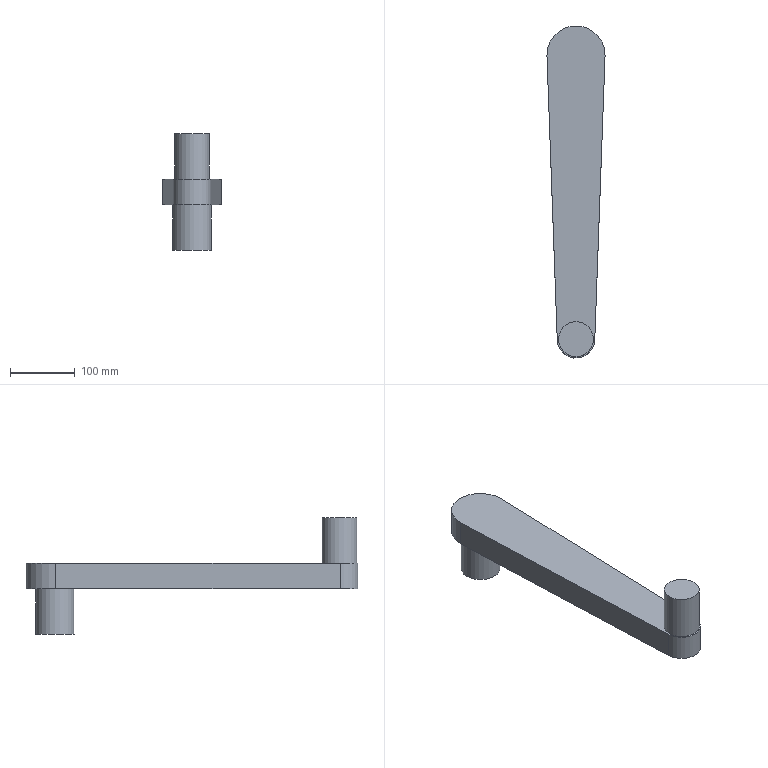Component | NX | PART_3 | 1 solid | 10 faces | box 90 x 514.09 x 180 mm | volume 1841830 mm3 | plane 6 | cylinder 4 | commonest cylinder face diameters 58 x1 90 x1 54 x1 60 x1
STEP:
#1=CARTESIAN_POINT('',(0.,0.,0.));
#2=DIRECTION('',(0.,0.,1.));
#3=DIRECTION('',(1.,0.,0.));
#4=AXIS2_PLACEMENT_3D('',#1,#2,#3);
#5=CARTESIAN_POINT('',(-201.014,-230.518,0.));
#6=VERTEX_POINT('',#5);
#7=CARTESIAN_POINT('',(-185.024,-670.023,0.));
#8=VERTEX_POINT('',#7);
#9=CARTESIAN_POINT('',(-201.014,-230.518,0.));
#10=DIRECTION('',(0.03636,-0.9993,0.));
#11=VECTOR('',#10,1.);
#12=LINE('',#9,#11);
#13=CARTESIAN_POINT('',(-201.014,-230.518,40.));
#14=DIRECTION('',(0.9993,0.03636,0.));
#15=DIRECTION('',(-0.03636,0.9993,0.));
#16=AXIS2_PLACEMENT_3D('',#13,#14,#15);
#17=PLANE('',#16);
#18=CARTESIAN_POINT('',(0.,-40.));
#19=DIRECTION('',(-1.,0.));
#20=VECTOR('',#19,1.);
#21=LINE('',#18,#20);
#22=(GEOMETRIC_REPRESENTATION_CONTEXT(2)PARAMETRIC_REPRESENTATION_CONTEXT()REPRESENTATION_CONTEXT('',''));
#23=DEFINITIONAL_REPRESENTATION('',(#21),#22);
#24=PCURVE('',#17,#23);
#25=CARTESIAN_POINT('',(-156.043,-668.969,0.));
#26=DIRECTION('',(0.,0.,1.));
#27=DIRECTION('',(1.,0.,0.));
#28=AXIS2_PLACEMENT_3D('',#25,#26,#27);
#29=PLANE('',#28);
#30=CARTESIAN_POINT('',(-44.97,438.451));
#31=DIRECTION('',(0.03636,-0.9993));
#32=VECTOR('',#31,1.);
#33=LINE('',#30,#32);
#34=(GEOMETRIC_REPRESENTATION_CONTEXT(2)PARAMETRIC_REPRESENTATION_CONTEXT()REPRESENTATION_CONTEXT('',''));
#35=DEFINITIONAL_REPRESENTATION('',(#33),#34);
#36=PCURVE('',#29,#35);
#37=SURFACE_CURVE('',#12,(#24,#36),.PCURVE_S1.);
#38=EDGE_CURVE('',#6,#8,#37,.T.);
#39=ORIENTED_EDGE('',*,*,#38,.T.);
#40=CARTESIAN_POINT('',(-185.024,-670.023,40.));
#41=VERTEX_POINT('',#40);
#42=CARTESIAN_POINT('',(-185.024,-670.023,40.));
#43=DIRECTION('',(0.,0.,-1.));
#44=VECTOR('',#43,1.);
#45=LINE('',#42,#44);
#46=CARTESIAN_POINT('',(-439.796,0.));
#47=DIRECTION('',(0.,-1.));
#48=VECTOR('',#47,1.);
#49=LINE('',#46,#48);
#50=(GEOMETRIC_REPRESENTATION_CONTEXT(2)PARAMETRIC_REPRESENTATION_CONTEXT()REPRESENTATION_CONTEXT('',''));
#51=DEFINITIONAL_REPRESENTATION('',(#49),#50);
#52=PCURVE('',#17,#51);
#53=CARTESIAN_POINT('',(-156.043,-668.969,40.));
#54=DIRECTION('',(0.,0.,-1.));
#55=DIRECTION('',(-1.,0.,0.));
#56=AXIS2_PLACEMENT_3D('',#53,#54,#55);
#57=CYLINDRICAL_SURFACE('',#56,29.);
#58=CARTESIAN_POINT('',(6.247,0.));
#59=DIRECTION('',(0.,1.));
#60=VECTOR('',#59,1.);
#61=LINE('',#58,#60);
#62=(GEOMETRIC_REPRESENTATION_CONTEXT(2)PARAMETRIC_REPRESENTATION_CONTEXT()REPRESENTATION_CONTEXT('',''));
#63=DEFINITIONAL_REPRESENTATION('',(#61),#62);
#64=PCURVE('',#57,#63);
#65=SURFACE_CURVE('',#45,(#52,#64),.PCURVE_S1.);
#66=EDGE_CURVE('',#41,#8,#65,.T.);
#67=ORIENTED_EDGE('',*,*,#66,.F.);
#68=CARTESIAN_POINT('',(-201.014,-230.518,40.));
#69=VERTEX_POINT('',#68);
#70=CARTESIAN_POINT('',(-201.014,-230.518,40.));
#71=DIRECTION('',(0.03636,-0.9993,0.));
#72=VECTOR('',#71,1.);
#73=LINE('',#70,#72);
#74=CARTESIAN_POINT('',(0.,0.));
#75=DIRECTION('',(-1.,0.));
#76=VECTOR('',#75,1.);
#77=LINE('',#74,#76);
#78=(GEOMETRIC_REPRESENTATION_CONTEXT(2)PARAMETRIC_REPRESENTATION_CONTEXT()REPRESENTATION_CONTEXT('',''));
#79=DEFINITIONAL_REPRESENTATION('',(#77),#78);
#80=PCURVE('',#17,#79);
#81=CARTESIAN_POINT('',(-156.043,-668.969,40.));
#82=DIRECTION('',(0.,0.,1.));
#83=DIRECTION('',(1.,0.,0.));
#84=AXIS2_PLACEMENT_3D('',#81,#82,#83);
#85=PLANE('',#84);
#86=CARTESIAN_POINT('',(-44.97,438.451));
#87=DIRECTION('',(0.03636,-0.9993));
#88=VECTOR('',#87,1.);
#89=LINE('',#86,#88);
#90=(GEOMETRIC_REPRESENTATION_CONTEXT(2)PARAMETRIC_REPRESENTATION_CONTEXT()REPRESENTATION_CONTEXT('',''));
#91=DEFINITIONAL_REPRESENTATION('',(#89),#90);
#92=PCURVE('',#85,#91);
#93=SURFACE_CURVE('',#73,(#80,#92),.PCURVE_S1.);
#94=EDGE_CURVE('',#69,#41,#93,.T.);
#95=ORIENTED_EDGE('',*,*,#94,.F.);
#96=CARTESIAN_POINT('',(-201.014,-230.518,40.));
#97=DIRECTION('',(0.,0.,-1.));
#98=VECTOR('',#97,1.);
#99=LINE('',#96,#98);
#100=CARTESIAN_POINT('',(0.,0.));
#101=DIRECTION('',(0.,-1.));
#102=VECTOR('',#101,1.);
#103=LINE('',#100,#102);
#104=(GEOMETRIC_REPRESENTATION_CONTEXT(2)PARAMETRIC_REPRESENTATION_CONTEXT()REPRESENTATION_CONTEXT('',''));
#105=DEFINITIONAL_REPRESENTATION('',(#103),#104);
#106=PCURVE('',#17,#105);
#107=CARTESIAN_POINT('',(-156.043,-228.882,40.));
#108=DIRECTION('',(0.,0.,-1.));
#109=DIRECTION('',(-1.,0.,0.));
#110=AXIS2_PLACEMENT_3D('',#107,#108,#109);
#111=CYLINDRICAL_SURFACE('',#110,45.);
#112=CARTESIAN_POINT('',(-0.03636,0.));
#113=DIRECTION('',(0.,1.));
#114=VECTOR('',#113,1.);
#115=LINE('',#112,#114);
#116=(GEOMETRIC_REPRESENTATION_CONTEXT(2)PARAMETRIC_REPRESENTATION_CONTEXT()REPRESENTATION_CONTEXT('',''));
#117=DEFINITIONAL_REPRESENTATION('',(#115),#116);
#118=PCURVE('',#111,#117);
#119=SURFACE_CURVE('',#99,(#106,#118),.PCURVE_S1.);
#120=EDGE_CURVE('',#69,#6,#119,.T.);
#121=ORIENTED_EDGE('',*,*,#120,.T.);
#122=EDGE_LOOP('',(#39,#67,#95,#121));
#123=FACE_BOUND('',#122,.T.);
#124=ADVANCED_FACE('',(#123),#17,.F.);
#125=CARTESIAN_POINT('',(-127.062,-670.023,0.));
#126=VERTEX_POINT('',#125);
#127=CARTESIAN_POINT('',(-156.043,-668.969,0.));
#128=DIRECTION('',(0.,0.,1.));
#129=DIRECTION('',(1.,0.,0.));
#130=AXIS2_PLACEMENT_3D('',#127,#128,#129);
#131=CIRCLE('',#130,29.);
#132=CARTESIAN_POINT('',(9.425,40.));
#133=DIRECTION('',(-1.,0.));
#134=VECTOR('',#133,1.);
#135=LINE('',#132,#134);
#136=(GEOMETRIC_REPRESENTATION_CONTEXT(2)PARAMETRIC_REPRESENTATION_CONTEXT()REPRESENTATION_CONTEXT('',''));
#137=DEFINITIONAL_REPRESENTATION('',(#135),#136);
#138=PCURVE('',#57,#137);
#139=CARTESIAN_POINT('',(0.,0.));
#140=DIRECTION('',(1.,0.));
#141=AXIS2_PLACEMENT_2D('',#139,#140);
#142=CIRCLE('',#141,29.);
#143=(GEOMETRIC_REPRESENTATION_CONTEXT(2)PARAMETRIC_REPRESENTATION_CONTEXT()REPRESENTATION_CONTEXT('',''));
#144=DEFINITIONAL_REPRESENTATION('',(#142),#143);
#145=PCURVE('',#29,#144);
#146=SURFACE_CURVE('',#131,(#138,#145),.PCURVE_S1.);
#147=EDGE_CURVE('',#8,#126,#146,.T.);
#148=ORIENTED_EDGE('',*,*,#147,.T.);
#149=CARTESIAN_POINT('',(-127.062,-670.023,40.));
#150=VERTEX_POINT('',#149);
#151=CARTESIAN_POINT('',(-127.062,-670.023,40.));
#152=DIRECTION('',(0.,0.,-1.));
#153=VECTOR('',#152,1.);
#154=LINE('',#151,#153);
#155=CARTESIAN_POINT('',(3.178,0.));
#156=DIRECTION('',(0.,1.));
#157=VECTOR('',#156,1.);
#158=LINE('',#155,#157);
#159=(GEOMETRIC_REPRESENTATION_CONTEXT(2)PARAMETRIC_REPRESENTATION_CONTEXT()REPRESENTATION_CONTEXT('',''));
#160=DEFINITIONAL_REPRESENTATION('',(#158),#159);
#161=PCURVE('',#57,#160);
#162=CARTESIAN_POINT('',(-127.062,-670.023,40.));
#163=DIRECTION('',(-0.9993,0.03636,0.));
#164=DIRECTION('',(-0.03636,-0.9993,0.));
#165=AXIS2_PLACEMENT_3D('',#162,#163,#164);
#166=PLANE('',#165);
#167=CARTESIAN_POINT('',(0.,0.));
#168=DIRECTION('',(0.,-1.));
#169=VECTOR('',#168,1.);
#170=LINE('',#167,#169);
#171=(GEOMETRIC_REPRESENTATION_CONTEXT(2)PARAMETRIC_REPRESENTATION_CONTEXT()REPRESENTATION_CONTEXT('',''));
#172=DEFINITIONAL_REPRESENTATION('',(#170),#171);
#173=PCURVE('',#166,#172);
#174=SURFACE_CURVE('',#154,(#161,#173),.PCURVE_S1.);
#175=EDGE_CURVE('',#150,#126,#174,.T.);
#176=ORIENTED_EDGE('',*,*,#175,.F.);
#177=CARTESIAN_POINT('',(-156.043,-668.969,40.));
#178=DIRECTION('',(0.,0.,1.));
#179=DIRECTION('',(1.,0.,0.));
#180=AXIS2_PLACEMENT_3D('',#177,#178,#179);
#181=CIRCLE('',#180,29.);
#182=CARTESIAN_POINT('',(9.425,0.));
#183=DIRECTION('',(-1.,0.));
#184=VECTOR('',#183,1.);
#185=LINE('',#182,#184);
#186=(GEOMETRIC_REPRESENTATION_CONTEXT(2)PARAMETRIC_REPRESENTATION_CONTEXT()REPRESENTATION_CONTEXT('',''));
#187=DEFINITIONAL_REPRESENTATION('',(#185),#186);
#188=PCURVE('',#57,#187);
#189=CARTESIAN_POINT('',(0.,0.));
#190=DIRECTION('',(1.,0.));
#191=AXIS2_PLACEMENT_2D('',#189,#190);
#192=CIRCLE('',#191,29.);
#193=(GEOMETRIC_REPRESENTATION_CONTEXT(2)PARAMETRIC_REPRESENTATION_CONTEXT()REPRESENTATION_CONTEXT('',''));
#194=DEFINITIONAL_REPRESENTATION('',(#192),#193);
#195=PCURVE('',#85,#194);
#196=SURFACE_CURVE('',#181,(#188,#195),.PCURVE_S1.);
#197=EDGE_CURVE('',#41,#150,#196,.T.);
#198=ORIENTED_EDGE('',*,*,#197,.F.);
#199=ORIENTED_EDGE('',*,*,#66,.T.);
#200=EDGE_LOOP('',(#148,#176,#198,#199));
#201=FACE_BOUND('',#200,.T.);
#202=ADVANCED_FACE('',(#201),#57,.T.);
#203=CARTESIAN_POINT('',(-111.073,-230.518,0.));
#204=VERTEX_POINT('',#203);
#205=CARTESIAN_POINT('',(-127.062,-670.023,0.));
#206=DIRECTION('',(0.03636,0.9993,0.));
#207=VECTOR('',#206,1.);
#208=LINE('',#205,#207);
#209=CARTESIAN_POINT('',(0.,-40.));
#210=DIRECTION('',(-1.,0.));
#211=VECTOR('',#210,1.);
#212=LINE('',#209,#211);
#213=(GEOMETRIC_REPRESENTATION_CONTEXT(2)PARAMETRIC_REPRESENTATION_CONTEXT()REPRESENTATION_CONTEXT('',''));
#214=DEFINITIONAL_REPRESENTATION('',(#212),#213);
#215=PCURVE('',#166,#214);
#216=CARTESIAN_POINT('',(28.981,-1.054));
#217=DIRECTION('',(0.03636,0.9993));
#218=VECTOR('',#217,1.);
#219=LINE('',#216,#218);
#220=(GEOMETRIC_REPRESENTATION_CONTEXT(2)PARAMETRIC_REPRESENTATION_CONTEXT()REPRESENTATION_CONTEXT('',''));
#221=DEFINITIONAL_REPRESENTATION('',(#219),#220);
#222=PCURVE('',#29,#221);
#223=SURFACE_CURVE('',#208,(#215,#222),.PCURVE_S1.);
#224=EDGE_CURVE('',#126,#204,#223,.T.);
#225=ORIENTED_EDGE('',*,*,#224,.T.);
#226=CARTESIAN_POINT('',(-111.073,-230.518,40.));
#227=VERTEX_POINT('',#226);
#228=CARTESIAN_POINT('',(-111.073,-230.518,40.));
#229=DIRECTION('',(0.,0.,-1.));
#230=VECTOR('',#229,1.);
#231=LINE('',#228,#230);
#232=CARTESIAN_POINT('',(-439.796,0.));
#233=DIRECTION('',(0.,-1.));
#234=VECTOR('',#233,1.);
#235=LINE('',#232,#234);
#236=(GEOMETRIC_REPRESENTATION_CONTEXT(2)PARAMETRIC_REPRESENTATION_CONTEXT()REPRESENTATION_CONTEXT('',''));
#237=DEFINITIONAL_REPRESENTATION('',(#235),#236);
#238=PCURVE('',#166,#237);
#239=CARTESIAN_POINT('',(3.178,0.));
#240=DIRECTION('',(0.,1.));
#241=VECTOR('',#240,1.);
#242=LINE('',#239,#241);
#243=(GEOMETRIC_REPRESENTATION_CONTEXT(2)PARAMETRIC_REPRESENTATION_CONTEXT()REPRESENTATION_CONTEXT('',''));
#244=DEFINITIONAL_REPRESENTATION('',(#242),#243);
#245=PCURVE('',#111,#244);
#246=SURFACE_CURVE('',#231,(#238,#245),.PCURVE_S1.);
#247=EDGE_CURVE('',#227,#204,#246,.T.);
#248=ORIENTED_EDGE('',*,*,#247,.F.);
#249=CARTESIAN_POINT('',(-127.062,-670.023,40.));
#250=DIRECTION('',(0.03636,0.9993,0.));
#251=VECTOR('',#250,1.);
#252=LINE('',#249,#251);
#253=CARTESIAN_POINT('',(0.,0.));
#254=DIRECTION('',(-1.,0.));
#255=VECTOR('',#254,1.);
#256=LINE('',#253,#255);
#257=(GEOMETRIC_REPRESENTATION_CONTEXT(2)PARAMETRIC_REPRESENTATION_CONTEXT()REPRESENTATION_CONTEXT('',''));
#258=DEFINITIONAL_REPRESENTATION('',(#256),#257);
#259=PCURVE('',#166,#258);
#260=CARTESIAN_POINT('',(28.981,-1.054));
#261=DIRECTION('',(0.03636,0.9993));
#262=VECTOR('',#261,1.);
#263=LINE('',#260,#262);
#264=(GEOMETRIC_REPRESENTATION_CONTEXT(2)PARAMETRIC_REPRESENTATION_CONTEXT()REPRESENTATION_CONTEXT('',''));
#265=DEFINITIONAL_REPRESENTATION('',(#263),#264);
#266=PCURVE('',#85,#265);
#267=SURFACE_CURVE('',#252,(#259,#266),.PCURVE_S1.);
#268=EDGE_CURVE('',#150,#227,#267,.T.);
#269=ORIENTED_EDGE('',*,*,#268,.F.);
#270=ORIENTED_EDGE('',*,*,#175,.T.);
#271=EDGE_LOOP('',(#225,#248,#269,#270));
#272=FACE_BOUND('',#271,.T.);
#273=ADVANCED_FACE('',(#272),#166,.F.);
#274=CARTESIAN_POINT('',(-156.043,-228.882,0.));
#275=DIRECTION('',(0.,0.,1.));
#276=DIRECTION('',(1.,0.,0.));
#277=AXIS2_PLACEMENT_3D('',#274,#275,#276);
#278=CIRCLE('',#277,45.);
#279=CARTESIAN_POINT('',(9.425,40.));
#280=DIRECTION('',(-1.,0.));
#281=VECTOR('',#280,1.);
#282=LINE('',#279,#281);
#283=(GEOMETRIC_REPRESENTATION_CONTEXT(2)PARAMETRIC_REPRESENTATION_CONTEXT()REPRESENTATION_CONTEXT('',''));
#284=DEFINITIONAL_REPRESENTATION('',(#282),#283);
#285=PCURVE('',#111,#284);
#286=CARTESIAN_POINT('',(0.,440.087));
#287=DIRECTION('',(1.,0.));
#288=AXIS2_PLACEMENT_2D('',#286,#287);
#289=CIRCLE('',#288,45.);
#290=(GEOMETRIC_REPRESENTATION_CONTEXT(2)PARAMETRIC_REPRESENTATION_CONTEXT()REPRESENTATION_CONTEXT('',''));
#291=DEFINITIONAL_REPRESENTATION('',(#289),#290);
#292=PCURVE('',#29,#291);
#293=SURFACE_CURVE('',#278,(#285,#292),.PCURVE_S1.);
#294=EDGE_CURVE('',#204,#6,#293,.T.);
#295=ORIENTED_EDGE('',*,*,#294,.T.);
#296=ORIENTED_EDGE('',*,*,#120,.F.);
#297=CARTESIAN_POINT('',(-156.043,-228.882,40.));
#298=DIRECTION('',(0.,0.,1.));
#299=DIRECTION('',(1.,0.,0.));
#300=AXIS2_PLACEMENT_3D('',#297,#298,#299);
#301=CIRCLE('',#300,45.);
#302=CARTESIAN_POINT('',(9.425,0.));
#303=DIRECTION('',(-1.,0.));
#304=VECTOR('',#303,1.);
#305=LINE('',#302,#304);
#306=(GEOMETRIC_REPRESENTATION_CONTEXT(2)PARAMETRIC_REPRESENTATION_CONTEXT()REPRESENTATION_CONTEXT('',''));
#307=DEFINITIONAL_REPRESENTATION('',(#305),#306);
#308=PCURVE('',#111,#307);
#309=CARTESIAN_POINT('',(0.,440.087));
#310=DIRECTION('',(1.,0.));
#311=AXIS2_PLACEMENT_2D('',#309,#310);
#312=CIRCLE('',#311,45.);
#313=(GEOMETRIC_REPRESENTATION_CONTEXT(2)PARAMETRIC_REPRESENTATION_CONTEXT()REPRESENTATION_CONTEXT('',''));
#314=DEFINITIONAL_REPRESENTATION('',(#312),#313);
#315=PCURVE('',#85,#314);
#316=SURFACE_CURVE('',#301,(#308,#315),.PCURVE_S1.);
#317=EDGE_CURVE('',#227,#69,#316,.T.);
#318=ORIENTED_EDGE('',*,*,#317,.F.);
#319=ORIENTED_EDGE('',*,*,#247,.T.);
#320=EDGE_LOOP('',(#295,#296,#318,#319));
#321=FACE_BOUND('',#320,.T.);
#322=ADVANCED_FACE('',(#321),#111,.T.);
#323=CARTESIAN_POINT('',(-129.043,-668.969,40.));
#324=VERTEX_POINT('',#323);
#325=CARTESIAN_POINT('',(-156.043,-668.969,40.));
#326=DIRECTION('',(0.,0.,1.));
#327=DIRECTION('',(1.,0.,0.));
#328=AXIS2_PLACEMENT_3D('',#325,#326,#327);
#329=CIRCLE('',#328,27.);
#330=CARTESIAN_POINT('',(0.,0.));
#331=DIRECTION('',(1.,0.));
#332=AXIS2_PLACEMENT_2D('',#330,#331);
#333=CIRCLE('',#332,27.);
#334=(GEOMETRIC_REPRESENTATION_CONTEXT(2)PARAMETRIC_REPRESENTATION_CONTEXT()REPRESENTATION_CONTEXT('',''));
#335=DEFINITIONAL_REPRESENTATION('',(#333),#334);
#336=PCURVE('',#85,#335);
#337=CARTESIAN_POINT('',(-156.043,-668.969,110.));
#338=DIRECTION('',(0.,0.,-1.));
#339=DIRECTION('',(-1.,0.,0.));
#340=AXIS2_PLACEMENT_3D('',#337,#338,#339);
#341=CYLINDRICAL_SURFACE('',#340,27.);
#342=CARTESIAN_POINT('',(9.425,70.));
#343=DIRECTION('',(-1.,0.));
#344=VECTOR('',#343,1.);
#345=LINE('',#342,#344);
#346=(GEOMETRIC_REPRESENTATION_CONTEXT(2)PARAMETRIC_REPRESENTATION_CONTEXT()REPRESENTATION_CONTEXT('',''));
#347=DEFINITIONAL_REPRESENTATION('',(#345),#346);
#348=PCURVE('',#341,#347);
#349=SURFACE_CURVE('',#329,(#336,#348),.PCURVE_S1.);
#350=EDGE_CURVE('',#324,#324,#349,.T.);
#351=ORIENTED_EDGE('',*,*,#350,.F.);
#352=EDGE_LOOP('',(#351));
#353=FACE_BOUND('',#352,.T.);
#354=ORIENTED_EDGE('',*,*,#94,.T.);
#355=ORIENTED_EDGE('',*,*,#197,.T.);
#356=ORIENTED_EDGE('',*,*,#268,.T.);
#357=ORIENTED_EDGE('',*,*,#317,.T.);
#358=EDGE_LOOP('',(#354,#355,#356,#357));
#359=FACE_BOUND('',#358,.T.);
#360=ADVANCED_FACE('',(#353,#359),#85,.T.);
#361=CARTESIAN_POINT('',(-126.043,-228.882,0.));
#362=VERTEX_POINT('',#361);
#363=CARTESIAN_POINT('',(-156.043,-228.882,0.));
#364=DIRECTION('',(0.,0.,-1.));
#365=DIRECTION('',(1.,0.,0.));
#366=AXIS2_PLACEMENT_3D('',#363,#364,#365);
#367=CIRCLE('',#366,30.);
#368=CARTESIAN_POINT('',(30.,440.087));
#369=CARTESIAN_POINT('',(30.,388.125));
#370=CARTESIAN_POINT('',(-15.,414.106));
#371=CARTESIAN_POINT('',(-60.,440.087));
#372=CARTESIAN_POINT('',(-15.,466.067));
#373=CARTESIAN_POINT('',(30.,492.048));
#374=CARTESIAN_POINT('',(30.,440.087));
#375=(BOUNDED_CURVE()B_SPLINE_CURVE(2,(#368,#369,#370,#371,#372,#373,#374),.UNSPECIFIED.,.T.,.F.)B_SPLINE_CURVE_WITH_KNOTS((1,2,2,2,2,1),(-2.094,0.,2.094,4.189,6.283,8.378),.UNSPECIFIED.)CURVE()GEOMETRIC_REPRESENTATION_ITEM()RATIONAL_B_SPLINE_CURVE((1.,0.5,1.,0.5,1.,0.5,1.))REPRESENTATION_ITEM(''));
#376=(GEOMETRIC_REPRESENTATION_CONTEXT(2)PARAMETRIC_REPRESENTATION_CONTEXT()REPRESENTATION_CONTEXT('',''));
#377=DEFINITIONAL_REPRESENTATION('',(#375),#376);
#378=PCURVE('',#29,#377);
#379=CARTESIAN_POINT('',(-156.043,-228.882,-70.));
#380=DIRECTION('',(0.,0.,1.));
#381=DIRECTION('',(1.,0.,0.));
#382=AXIS2_PLACEMENT_3D('',#379,#380,#381);
#383=CYLINDRICAL_SURFACE('',#382,30.);
#384=CARTESIAN_POINT('',(6.283,70.));
#385=DIRECTION('',(-1.,0.));
#386=VECTOR('',#385,1.);
#387=LINE('',#384,#386);
#388=(GEOMETRIC_REPRESENTATION_CONTEXT(2)PARAMETRIC_REPRESENTATION_CONTEXT()REPRESENTATION_CONTEXT('',''));
#389=DEFINITIONAL_REPRESENTATION('',(#387),#388);
#390=PCURVE('',#383,#389);
#391=SURFACE_CURVE('',#367,(#378,#390),.PCURVE_S1.);
#392=EDGE_CURVE('',#362,#362,#391,.T.);
#393=ORIENTED_EDGE('',*,*,#392,.F.);
#394=EDGE_LOOP('',(#393));
#395=FACE_BOUND('',#394,.T.);
#396=ORIENTED_EDGE('',*,*,#38,.F.);
#397=ORIENTED_EDGE('',*,*,#294,.F.);
#398=ORIENTED_EDGE('',*,*,#224,.F.);
#399=ORIENTED_EDGE('',*,*,#147,.F.);
#400=EDGE_LOOP('',(#396,#397,#398,#399));
#401=FACE_BOUND('',#400,.T.);
#402=ADVANCED_FACE('',(#395,#401),#29,.F.);
#403=CARTESIAN_POINT('',(-129.043,-668.969,110.));
#404=VERTEX_POINT('',#403);
#405=CARTESIAN_POINT('',(-156.043,-668.969,110.));
#406=DIRECTION('',(0.,0.,1.));
#407=DIRECTION('',(1.,0.,0.));
#408=AXIS2_PLACEMENT_3D('',#405,#406,#407);
#409=CIRCLE('',#408,27.);
#410=CARTESIAN_POINT('',(9.425,0.));
#411=DIRECTION('',(-1.,0.));
#412=VECTOR('',#411,1.);
#413=LINE('',#410,#412);
#414=(GEOMETRIC_REPRESENTATION_CONTEXT(2)PARAMETRIC_REPRESENTATION_CONTEXT()REPRESENTATION_CONTEXT('',''));
#415=DEFINITIONAL_REPRESENTATION('',(#413),#414);
#416=PCURVE('',#341,#415);
#417=CARTESIAN_POINT('',(-156.043,-668.969,110.));
#418=DIRECTION('',(0.,0.,1.));
#419=DIRECTION('',(1.,0.,0.));
#420=AXIS2_PLACEMENT_3D('',#417,#418,#419);
#421=PLANE('',#420);
#422=CARTESIAN_POINT('',(0.,0.));
#423=DIRECTION('',(1.,0.));
#424=AXIS2_PLACEMENT_2D('',#422,#423);
#425=CIRCLE('',#424,27.);
#426=(GEOMETRIC_REPRESENTATION_CONTEXT(2)PARAMETRIC_REPRESENTATION_CONTEXT()REPRESENTATION_CONTEXT('',''));
#427=DEFINITIONAL_REPRESENTATION('',(#425),#426);
#428=PCURVE('',#421,#427);
#429=SURFACE_CURVE('',#409,(#416,#428),.PCURVE_S1.);
#430=EDGE_CURVE('',#404,#404,#429,.T.);
#431=ORIENTED_EDGE('',*,*,#430,.F.);
#432=CARTESIAN_POINT('',(-129.043,-668.969,110.));
#433=CARTESIAN_POINT('',(-129.043,-668.969,40.));
#434=B_SPLINE_CURVE_WITH_KNOTS('',1,(#432,#433),.UNSPECIFIED.,.F.,.F.,(2,2),(0.,70.),.PIECEWISE_BEZIER_KNOTS.);
#435=CARTESIAN_POINT('',(9.425,0.));
#436=DIRECTION('',(0.,1.));
#437=VECTOR('',#436,1.);
#438=LINE('',#435,#437);
#439=(GEOMETRIC_REPRESENTATION_CONTEXT(2)PARAMETRIC_REPRESENTATION_CONTEXT()REPRESENTATION_CONTEXT('',''));
#440=DEFINITIONAL_REPRESENTATION('',(#438),#439);
#441=PCURVE('',#341,#440);
#442=CARTESIAN_POINT('',(3.142,0.));
#443=DIRECTION('',(0.,1.));
#444=VECTOR('',#443,1.);
#445=LINE('',#442,#444);
#446=(GEOMETRIC_REPRESENTATION_CONTEXT(2)PARAMETRIC_REPRESENTATION_CONTEXT()REPRESENTATION_CONTEXT('',''));
#447=DEFINITIONAL_REPRESENTATION('',(#445),#446);
#448=PCURVE('',#341,#447);
#449=SEAM_CURVE('',#434,(#441,#448),.PCURVE_S1.);
#450=EDGE_CURVE('',#404,#324,#449,.T.);
#451=ORIENTED_EDGE('',*,*,#450,.T.);
#452=ORIENTED_EDGE('',*,*,#350,.T.);
#453=ORIENTED_EDGE('',*,*,#450,.F.);
#454=EDGE_LOOP('',(#431,#451,#452,#453));
#455=FACE_BOUND('',#454,.T.);
#456=ADVANCED_FACE('',(#455),#341,.T.);
#457=ORIENTED_EDGE('',*,*,#430,.T.);
#458=EDGE_LOOP('',(#457));
#459=FACE_BOUND('',#458,.T.);
#460=ADVANCED_FACE('',(#459),#421,.T.);
#461=CARTESIAN_POINT('',(-126.043,-228.882,-70.));
#462=VERTEX_POINT('',#461);
#463=CARTESIAN_POINT('',(-156.043,-228.882,-70.));
#464=DIRECTION('',(0.,0.,-1.));
#465=DIRECTION('',(1.,0.,0.));
#466=AXIS2_PLACEMENT_3D('',#463,#464,#465);
#467=CIRCLE('',#466,30.);
#468=CARTESIAN_POINT('',(6.283,0.));
#469=DIRECTION('',(-1.,0.));
#470=VECTOR('',#469,1.);
#471=LINE('',#468,#470);
#472=(GEOMETRIC_REPRESENTATION_CONTEXT(2)PARAMETRIC_REPRESENTATION_CONTEXT()REPRESENTATION_CONTEXT('',''));
#473=DEFINITIONAL_REPRESENTATION('',(#471),#472);
#474=PCURVE('',#383,#473);
#475=CARTESIAN_POINT('',(-156.043,-228.882,-70.));
#476=DIRECTION('',(0.,0.,-1.));
#477=DIRECTION('',(-1.,0.,0.));
#478=AXIS2_PLACEMENT_3D('',#475,#476,#477);
#479=PLANE('',#478);
#480=CARTESIAN_POINT('',(0.,0.));
#481=DIRECTION('',(-1.,0.));
#482=AXIS2_PLACEMENT_2D('',#480,#481);
#483=CIRCLE('',#482,30.);
#484=(GEOMETRIC_REPRESENTATION_CONTEXT(2)PARAMETRIC_REPRESENTATION_CONTEXT()REPRESENTATION_CONTEXT('',''));
#485=DEFINITIONAL_REPRESENTATION('',(#483),#484);
#486=PCURVE('',#479,#485);
#487=SURFACE_CURVE('',#467,(#474,#486),.PCURVE_S1.);
#488=EDGE_CURVE('',#462,#462,#487,.T.);
#489=ORIENTED_EDGE('',*,*,#488,.F.);
#490=CARTESIAN_POINT('',(-126.043,-228.882,-70.));
#491=CARTESIAN_POINT('',(-126.043,-228.882,0.));
#492=B_SPLINE_CURVE_WITH_KNOTS('',1,(#490,#491),.UNSPECIFIED.,.F.,.F.,(2,2),(0.,70.),.PIECEWISE_BEZIER_KNOTS.);
#493=CARTESIAN_POINT('',(6.283,0.));
#494=DIRECTION('',(0.,1.));
#495=VECTOR('',#494,1.);
#496=LINE('',#493,#495);
#497=(GEOMETRIC_REPRESENTATION_CONTEXT(2)PARAMETRIC_REPRESENTATION_CONTEXT()REPRESENTATION_CONTEXT('',''));
#498=DEFINITIONAL_REPRESENTATION('',(#496),#497);
#499=PCURVE('',#383,#498);
#500=CARTESIAN_POINT('',(0.,0.));
#501=DIRECTION('',(0.,1.));
#502=VECTOR('',#501,1.);
#503=LINE('',#500,#502);
#504=(GEOMETRIC_REPRESENTATION_CONTEXT(2)PARAMETRIC_REPRESENTATION_CONTEXT()REPRESENTATION_CONTEXT('',''));
#505=DEFINITIONAL_REPRESENTATION('',(#503),#504);
#506=PCURVE('',#383,#505);
#507=SEAM_CURVE('',#492,(#499,#506),.PCURVE_S1.);
#508=EDGE_CURVE('',#462,#362,#507,.T.);
#509=ORIENTED_EDGE('',*,*,#508,.T.);
#510=ORIENTED_EDGE('',*,*,#392,.T.);
#511=ORIENTED_EDGE('',*,*,#508,.F.);
#512=EDGE_LOOP('',(#489,#509,#510,#511));
#513=FACE_BOUND('',#512,.T.);
#514=ADVANCED_FACE('',(#513),#383,.T.);
#515=ORIENTED_EDGE('',*,*,#488,.T.);
#516=EDGE_LOOP('',(#515));
#517=FACE_BOUND('',#516,.T.);
#518=ADVANCED_FACE('',(#517),#479,.T.);
#519=CLOSED_SHELL('',(#124,#202,#273,#322,#360,#402,#456,#460,#514,#518));
#520=MANIFOLD_SOLID_BREP('',#519);
#521=(LENGTH_UNIT()NAMED_UNIT(*)SI_UNIT(.MILLI.,.METRE.));
#522=UNCERTAINTY_MEASURE_WITH_UNIT(LENGTH_MEASURE(0.000002),#521,'','');
#523=(NAMED_UNIT(*)PLANE_ANGLE_UNIT()SI_UNIT($,.RADIAN.));
#524=(NAMED_UNIT(*)SI_UNIT($,.STERADIAN.)SOLID_ANGLE_UNIT());
#525=(GEOMETRIC_REPRESENTATION_CONTEXT(3)GLOBAL_UNCERTAINTY_ASSIGNED_CONTEXT((#522))GLOBAL_UNIT_ASSIGNED_CONTEXT((#521,#523,#524))REPRESENTATION_CONTEXT('',''));
#526=ADVANCED_BREP_SHAPE_REPRESENTATION('',(#4,#520),#525);